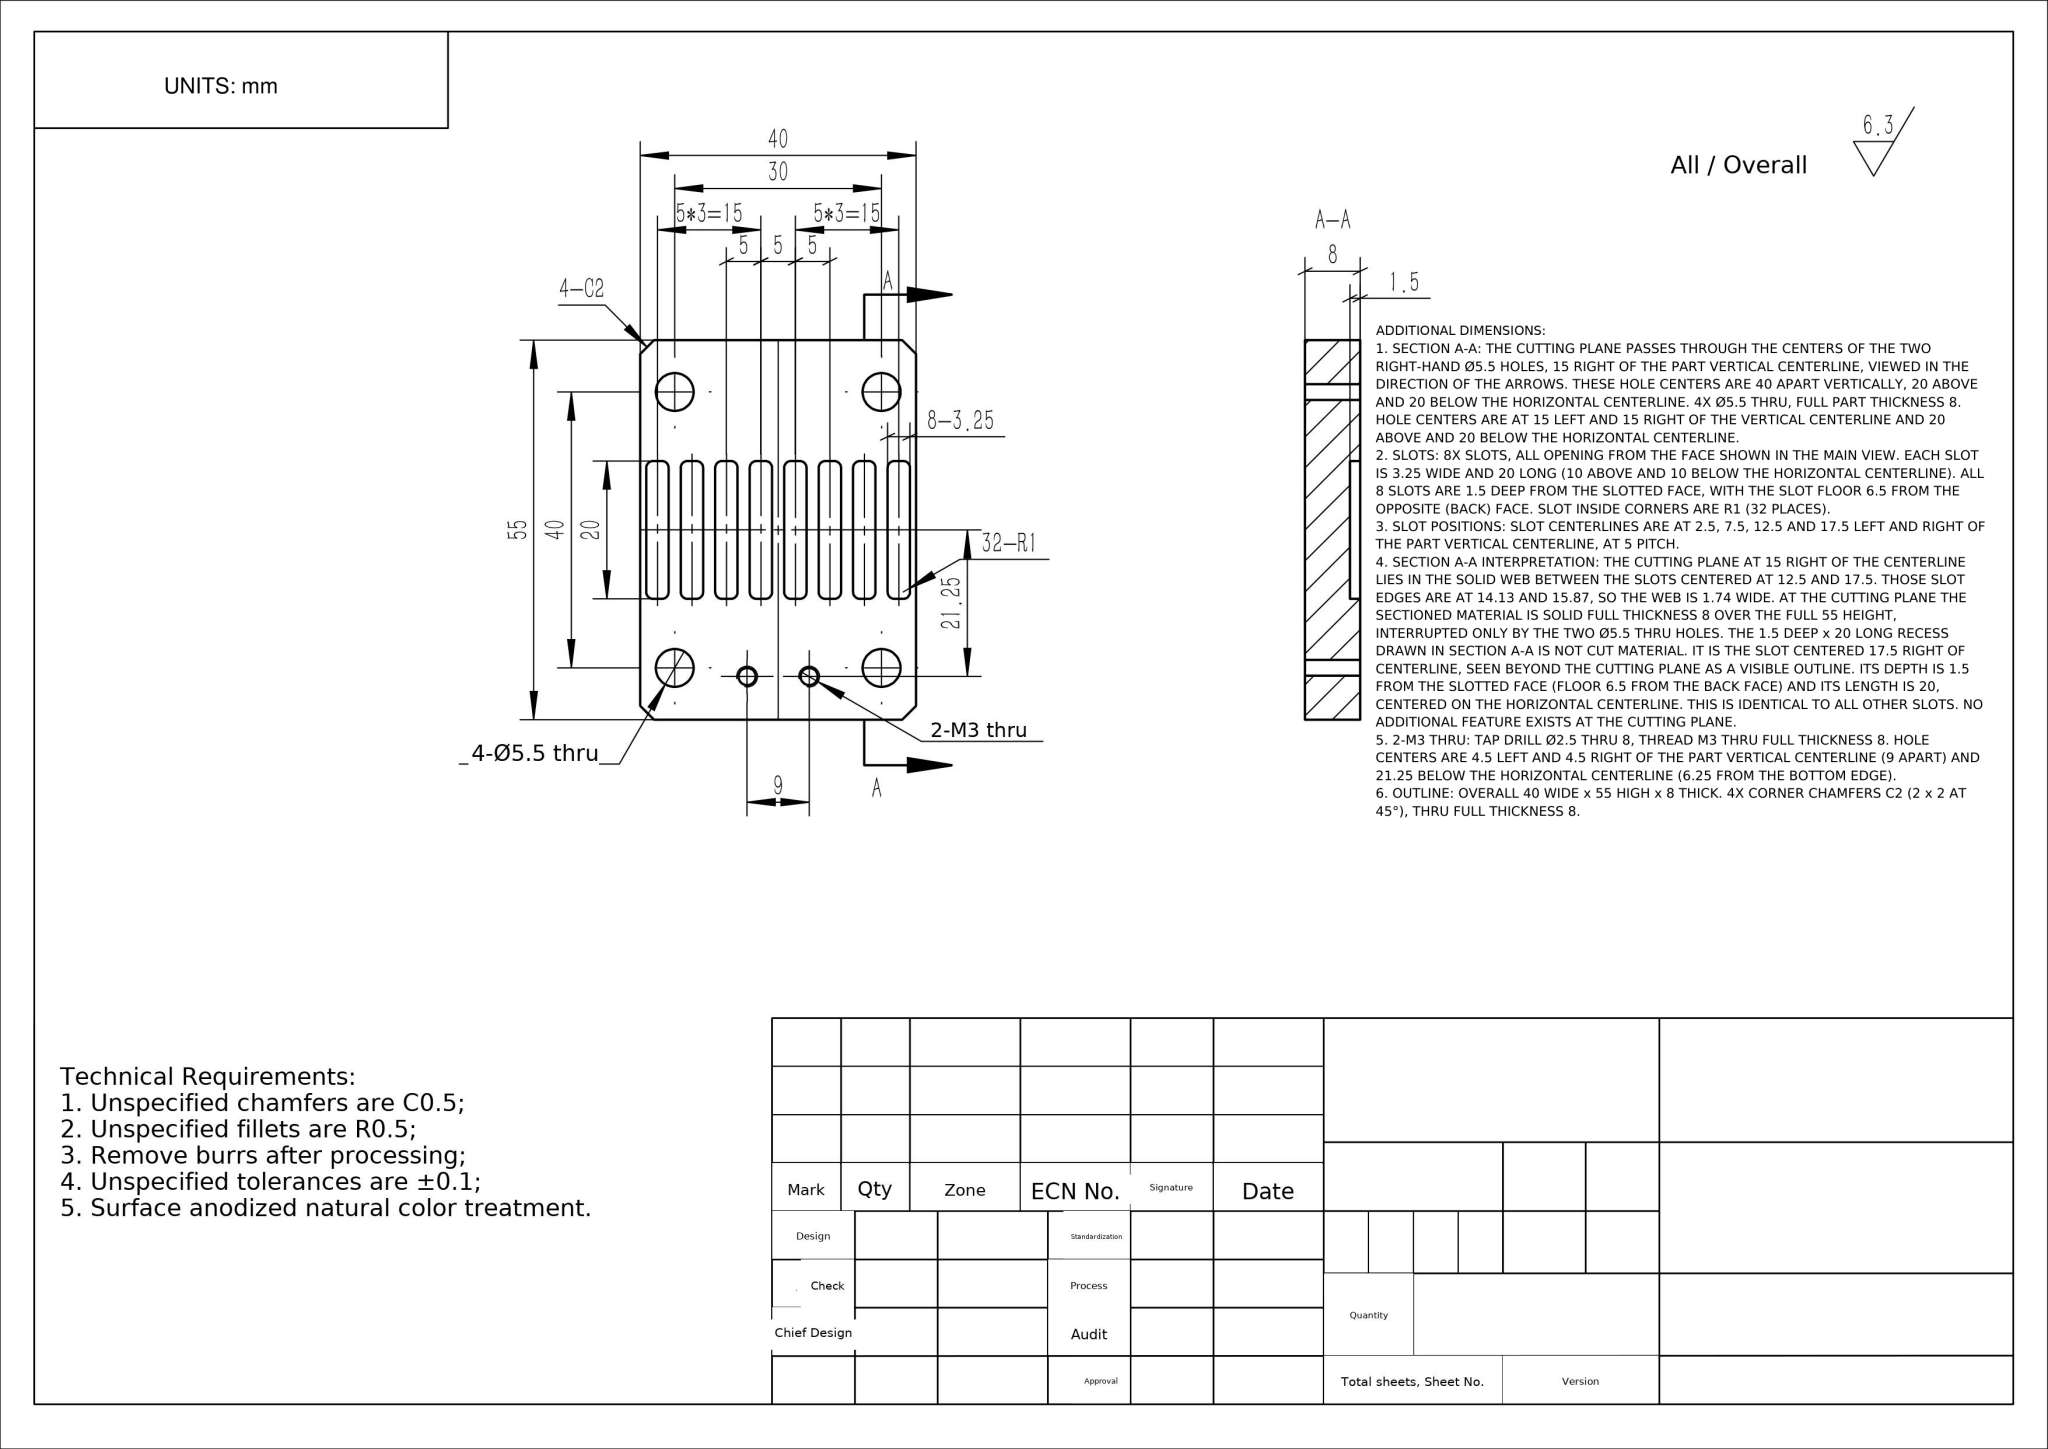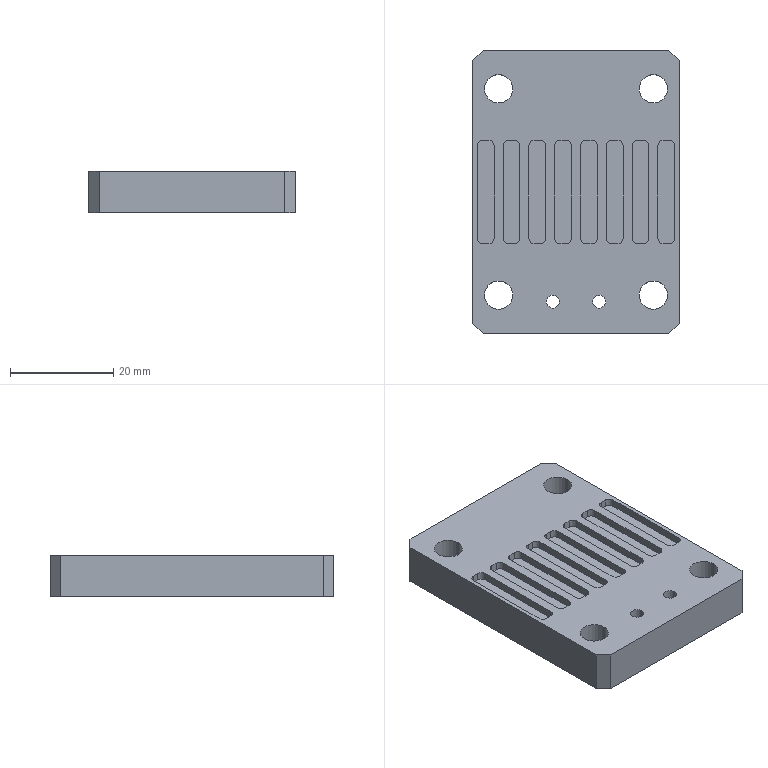Part | NX | mm | 1 solid | 94 faces | box 40 x 55 x 8 mm | volume 15927 mm3 | plane 50 | cylinder 44 | commonest cylinder face diameters 2 x32 5.5 x8 2.5 x4